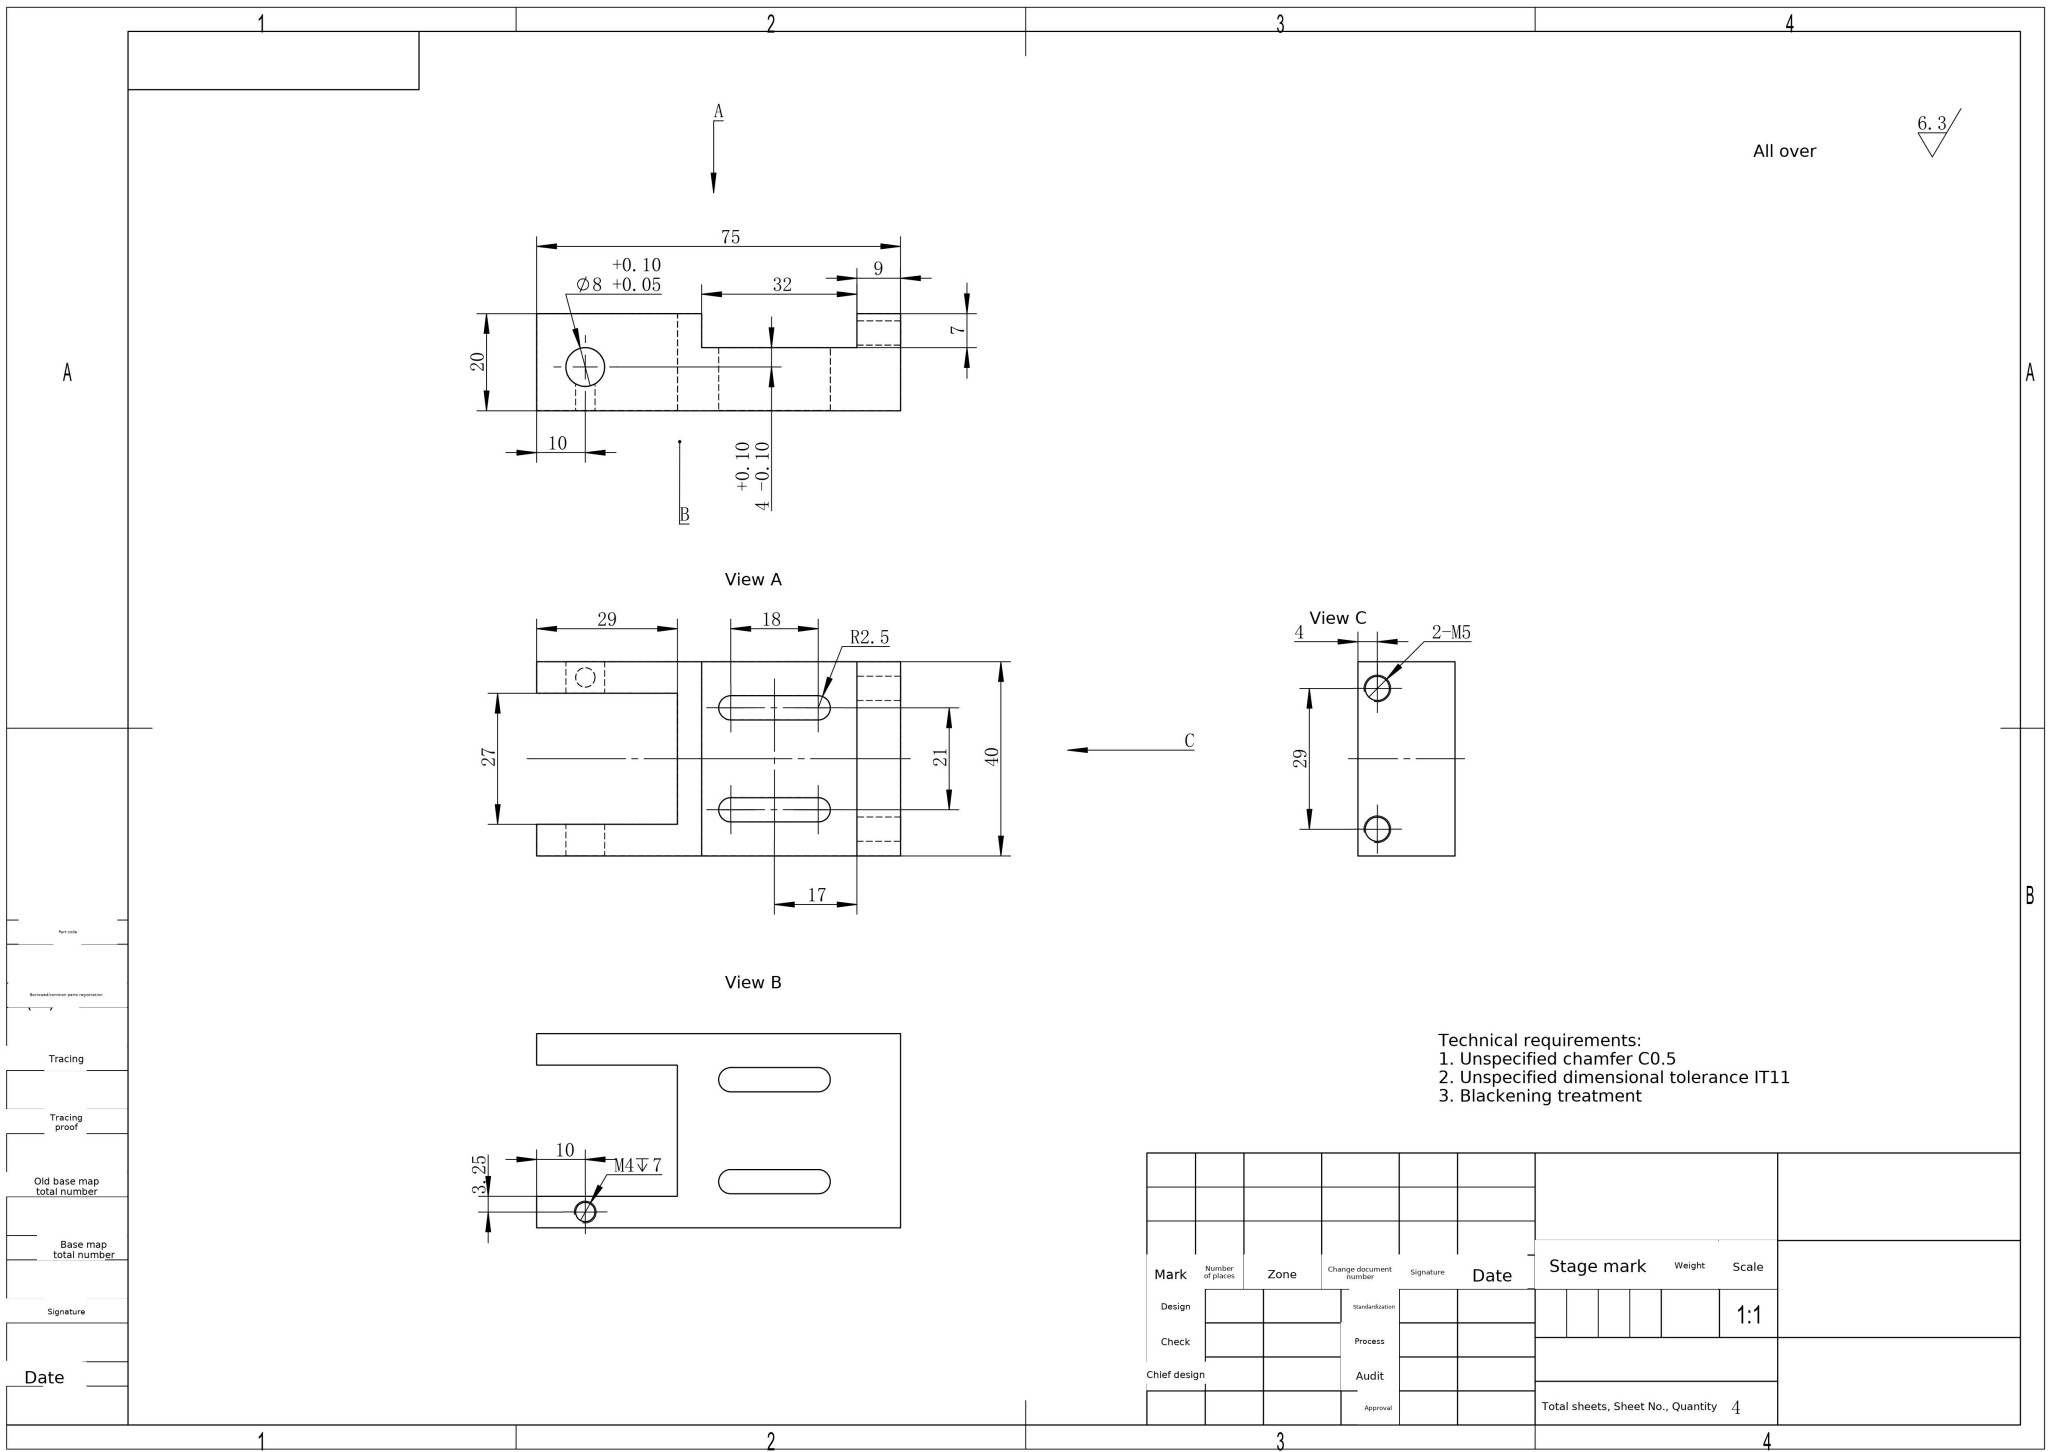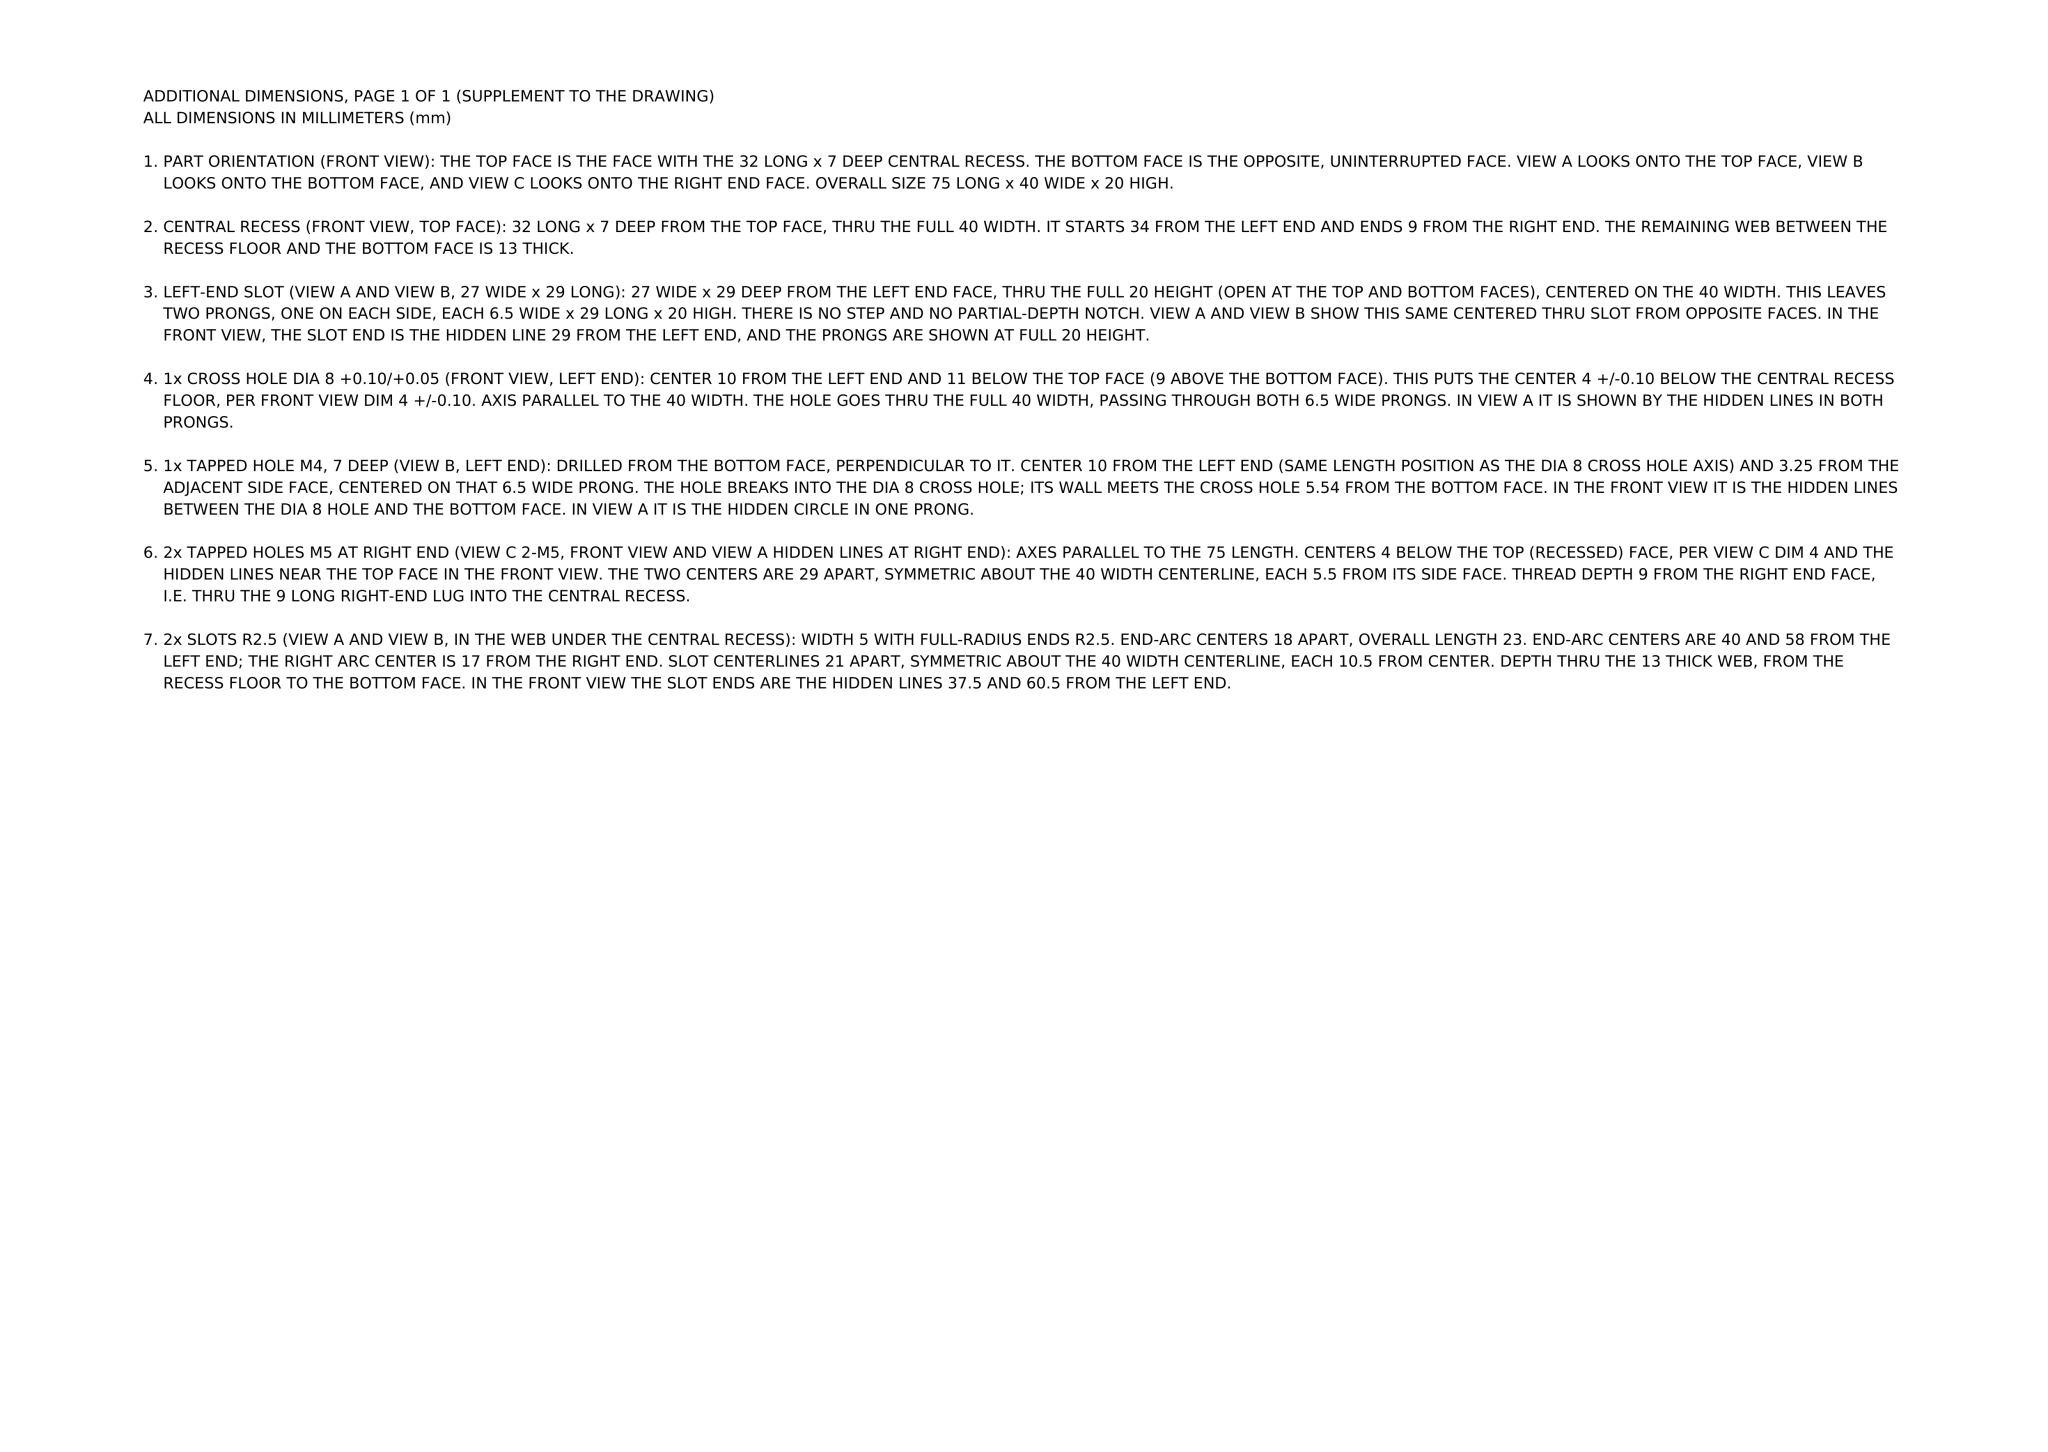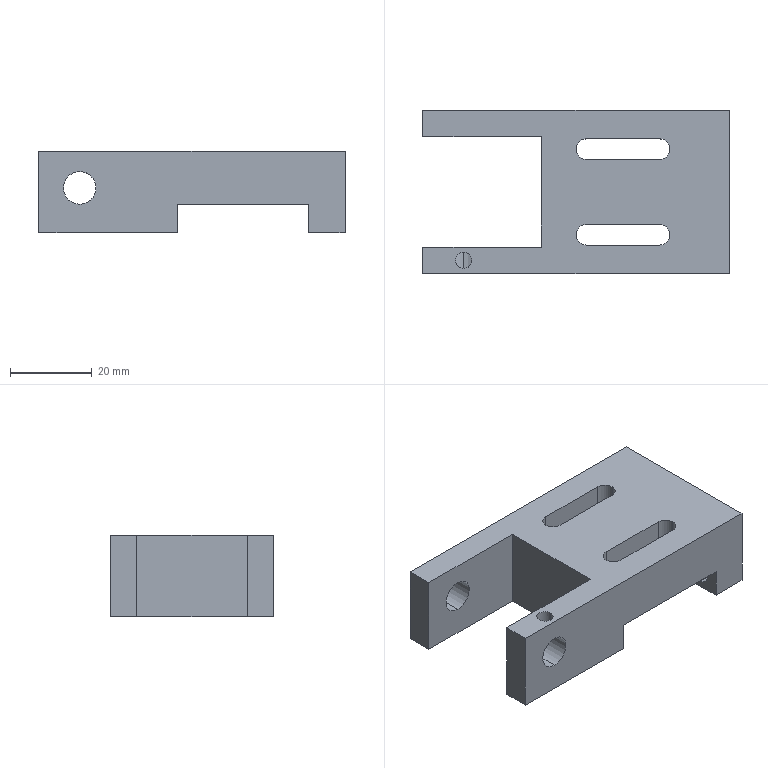Part | NX | mm | 1 solid | 36 faces | box 75 x 40 x 20 mm | volume 31458 mm3 | cylinder 18 | plane 18 | commonest cylinder face diameters 5 x12 8 x4 4 x2